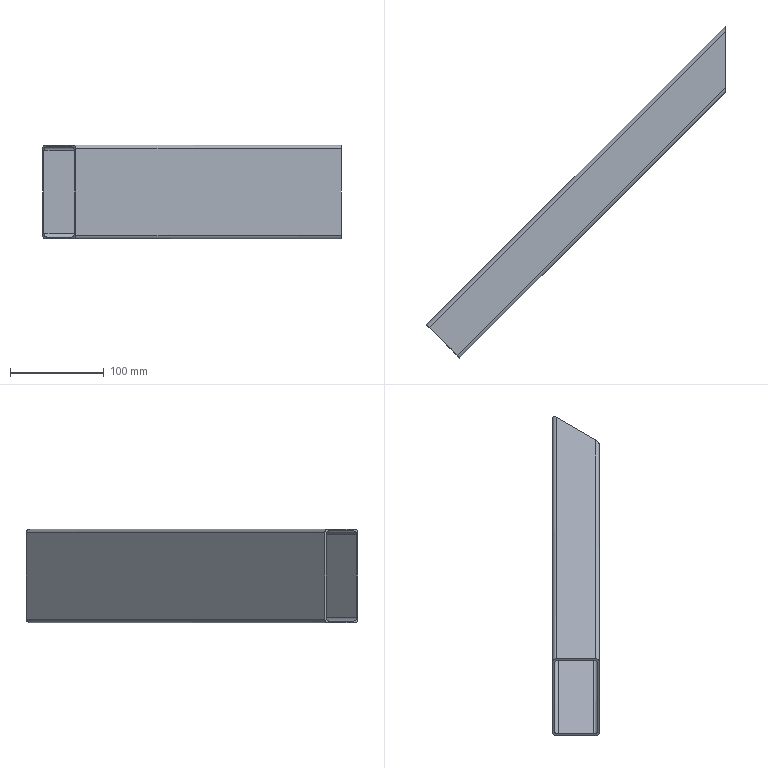Component | NX | SLID_FRAME_BEAM2 | 1 solid | 18 faces | volume 248200 mm3 | plane 10 | cylinder 8 | commonest cylinder face diameters 8 x8